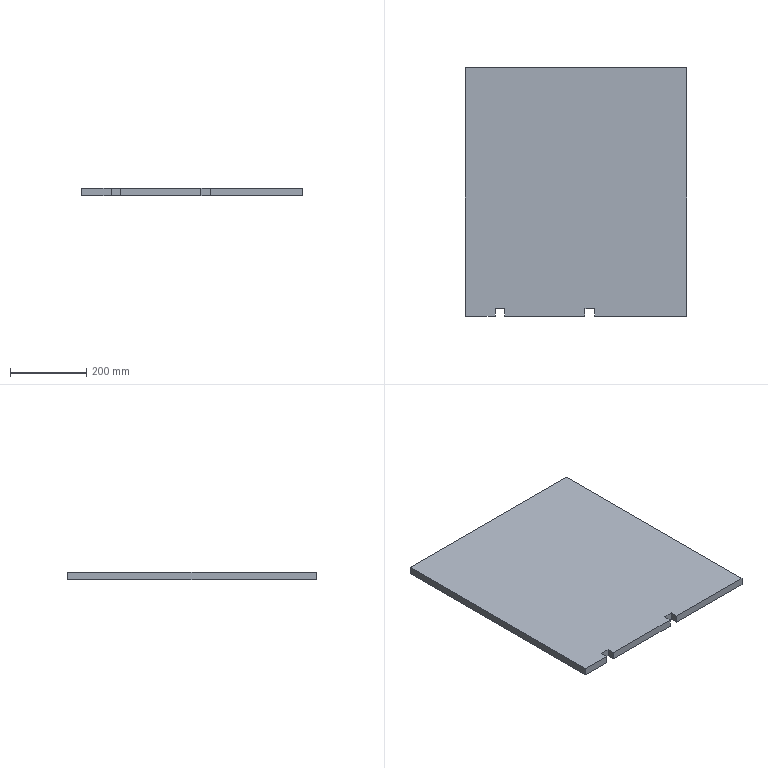Component | SolidWorks | ElectromagneticBeamBasePlate2-1 | 1 solid | 14 faces | box 579 x 650 x 20 mm | volume 7507000 mm3 | plane 14 | material Plain Carbon Steel
STEP:
#1=COLOUR_RGB('',0.7922,0.8196,0.9333);
#2=FILL_AREA_STYLE_COLOUR('',#1);
#3=FILL_AREA_STYLE('',(#2));
#4=SURFACE_STYLE_FILL_AREA(#3);
#5=SURFACE_SIDE_STYLE('',(#4));
#6=SURFACE_STYLE_USAGE(.BOTH.,#5);
#7=PRESENTATION_STYLE_ASSIGNMENT((#6));
#8=CARTESIAN_POINT('',(-258.877,140.226,239.923));
#9=VERTEX_POINT('',#8);
#10=CARTESIAN_POINT('',(-258.877,114.635,239.923));
#11=VERTEX_POINT('',#10);
#12=CARTESIAN_POINT('',(-258.877,140.226,239.923));
#13=DIRECTION('',(0.,-1.,-0.));
#14=VECTOR('',#13,39.37);
#15=LINE('',#12,#14);
#16=EDGE_CURVE('',#9,#11,#15,.T.);
#17=ORIENTED_EDGE('',*,*,#16,.F.);
#18=CARTESIAN_POINT('',(-258.877,140.226,239.136));
#19=VERTEX_POINT('',#18);
#20=CARTESIAN_POINT('',(-258.877,140.226,239.136));
#21=DIRECTION('',(0.,-0.,1.));
#22=VECTOR('',#21,39.37);
#23=LINE('',#20,#22);
#24=EDGE_CURVE('',#19,#9,#23,.T.);
#25=ORIENTED_EDGE('',*,*,#24,.F.);
#26=CARTESIAN_POINT('',(-258.877,114.635,239.136));
#27=VERTEX_POINT('',#26);
#28=CARTESIAN_POINT('',(-258.877,140.226,239.136));
#29=DIRECTION('',(0.,-1.,-0.));
#30=VECTOR('',#29,39.37);
#31=LINE('',#28,#30);
#32=EDGE_CURVE('',#19,#27,#31,.T.);
#33=ORIENTED_EDGE('',*,*,#32,.T.);
#34=CARTESIAN_POINT('',(-258.877,114.635,239.136));
#35=DIRECTION('',(0.,-0.,1.));
#36=VECTOR('',#35,39.37);
#37=LINE('',#34,#36);
#38=EDGE_CURVE('',#27,#11,#37,.T.);
#39=ORIENTED_EDGE('',*,*,#38,.T.);
#40=EDGE_LOOP('',(#17,#25,#33,#39));
#41=FACE_OUTER_BOUND('',#40,.T.);
#42=CARTESIAN_POINT('',(-258.877,140.226,239.136));
#43=DIRECTION('',(-1.,-0.,-0.));
#44=DIRECTION('',(0.,-1.,-0.));
#45=AXIS2_PLACEMENT_3D('',#42,#43,#44);
#46=PLANE('',#45);
#47=ADVANCED_FACE('',(#41),#46,.T.);
#48=CARTESIAN_POINT('',(-236.081,140.226,239.923));
#49=VERTEX_POINT('',#48);
#50=CARTESIAN_POINT('',(-258.877,140.226,239.923));
#51=DIRECTION('',(-1.,0.,0.));
#52=VECTOR('',#51,39.37);
#53=LINE('',#50,#52);
#54=EDGE_CURVE('',#49,#9,#53,.T.);
#55=ORIENTED_EDGE('',*,*,#54,.F.);
#56=CARTESIAN_POINT('',(-236.081,140.226,239.136));
#57=VERTEX_POINT('',#56);
#58=CARTESIAN_POINT('',(-236.081,140.226,239.136));
#59=DIRECTION('',(0.,-0.,1.));
#60=VECTOR('',#59,39.37);
#61=LINE('',#58,#60);
#62=EDGE_CURVE('',#57,#49,#61,.T.);
#63=ORIENTED_EDGE('',*,*,#62,.F.);
#64=CARTESIAN_POINT('',(-258.877,140.226,239.136));
#65=DIRECTION('',(-1.,0.,0.));
#66=VECTOR('',#65,39.37);
#67=LINE('',#64,#66);
#68=EDGE_CURVE('',#57,#19,#67,.T.);
#69=ORIENTED_EDGE('',*,*,#68,.T.);
#70=ORIENTED_EDGE('',*,*,#24,.T.);
#71=EDGE_LOOP('',(#55,#63,#69,#70));
#72=FACE_OUTER_BOUND('',#71,.T.);
#73=CARTESIAN_POINT('',(-258.877,140.226,239.136));
#74=DIRECTION('',(0.,1.,0.));
#75=DIRECTION('',(-1.,0.,0.));
#76=AXIS2_PLACEMENT_3D('',#73,#74,#75);
#77=PLANE('',#76);
#78=ADVANCED_FACE('',(#72),#77,.T.);
#79=CARTESIAN_POINT('',(-236.081,114.635,239.923));
#80=VERTEX_POINT('',#79);
#81=CARTESIAN_POINT('',(-236.081,140.226,239.923));
#82=DIRECTION('',(-0.,1.,0.));
#83=VECTOR('',#82,39.37);
#84=LINE('',#81,#83);
#85=EDGE_CURVE('',#80,#49,#84,.T.);
#86=ORIENTED_EDGE('',*,*,#85,.F.);
#87=CARTESIAN_POINT('',(-236.081,114.635,239.136));
#88=VERTEX_POINT('',#87);
#89=CARTESIAN_POINT('',(-236.081,114.635,239.136));
#90=DIRECTION('',(0.,-0.,1.));
#91=VECTOR('',#90,39.37);
#92=LINE('',#89,#91);
#93=EDGE_CURVE('',#88,#80,#92,.T.);
#94=ORIENTED_EDGE('',*,*,#93,.F.);
#95=CARTESIAN_POINT('',(-236.081,140.226,239.136));
#96=DIRECTION('',(-0.,1.,0.));
#97=VECTOR('',#96,39.37);
#98=LINE('',#95,#97);
#99=EDGE_CURVE('',#88,#57,#98,.T.);
#100=ORIENTED_EDGE('',*,*,#99,.T.);
#101=ORIENTED_EDGE('',*,*,#62,.T.);
#102=EDGE_LOOP('',(#86,#94,#100,#101));
#103=FACE_OUTER_BOUND('',#102,.T.);
#104=CARTESIAN_POINT('',(-236.081,140.226,239.136));
#105=DIRECTION('',(1.,0.,0.));
#106=DIRECTION('',(-0.,1.,0.));
#107=AXIS2_PLACEMENT_3D('',#104,#105,#106);
#108=PLANE('',#107);
#109=ADVANCED_FACE('',(#103),#108,.T.);
#110=CARTESIAN_POINT('',(-245.569,114.635,239.923));
#111=VERTEX_POINT('',#110);
#112=CARTESIAN_POINT('',(-245.569,114.635,239.923));
#113=DIRECTION('',(1.,0.,0.));
#114=VECTOR('',#113,39.37);
#115=LINE('',#112,#114);
#116=EDGE_CURVE('',#111,#80,#115,.T.);
#117=ORIENTED_EDGE('',*,*,#116,.F.);
#118=CARTESIAN_POINT('',(-245.569,114.635,239.136));
#119=VERTEX_POINT('',#118);
#120=CARTESIAN_POINT('',(-245.569,114.635,239.136));
#121=DIRECTION('',(0.,-0.,1.));
#122=VECTOR('',#121,39.37);
#123=LINE('',#120,#122);
#124=EDGE_CURVE('',#119,#111,#123,.T.);
#125=ORIENTED_EDGE('',*,*,#124,.F.);
#126=CARTESIAN_POINT('',(-245.569,114.635,239.136));
#127=DIRECTION('',(1.,0.,0.));
#128=VECTOR('',#127,39.37);
#129=LINE('',#126,#128);
#130=EDGE_CURVE('',#119,#88,#129,.T.);
#131=ORIENTED_EDGE('',*,*,#130,.T.);
#132=ORIENTED_EDGE('',*,*,#93,.T.);
#133=EDGE_LOOP('',(#117,#125,#131,#132));
#134=FACE_OUTER_BOUND('',#133,.T.);
#135=CARTESIAN_POINT('',(-245.569,114.635,239.136));
#136=DIRECTION('',(0.,-1.,-0.));
#137=DIRECTION('',(1.,0.,0.));
#138=AXIS2_PLACEMENT_3D('',#135,#136,#137);
#139=PLANE('',#138);
#140=ADVANCED_FACE('',(#134),#139,.T.);
#141=CARTESIAN_POINT('',(-245.569,115.423,239.923));
#142=VERTEX_POINT('',#141);
#143=CARTESIAN_POINT('',(-245.569,115.423,239.923));
#144=DIRECTION('',(0.,-1.,-0.));
#145=VECTOR('',#144,39.37);
#146=LINE('',#143,#145);
#147=EDGE_CURVE('',#142,#111,#146,.T.);
#148=ORIENTED_EDGE('',*,*,#147,.F.);
#149=CARTESIAN_POINT('',(-245.569,115.423,239.136));
#150=VERTEX_POINT('',#149);
#151=CARTESIAN_POINT('',(-245.569,115.423,239.136));
#152=DIRECTION('',(0.,-0.,1.));
#153=VECTOR('',#152,39.37);
#154=LINE('',#151,#153);
#155=EDGE_CURVE('',#150,#142,#154,.T.);
#156=ORIENTED_EDGE('',*,*,#155,.F.);
#157=CARTESIAN_POINT('',(-245.569,115.423,239.136));
#158=DIRECTION('',(0.,-1.,-0.));
#159=VECTOR('',#158,39.37);
#160=LINE('',#157,#159);
#161=EDGE_CURVE('',#150,#119,#160,.T.);
#162=ORIENTED_EDGE('',*,*,#161,.T.);
#163=ORIENTED_EDGE('',*,*,#124,.T.);
#164=EDGE_LOOP('',(#148,#156,#162,#163));
#165=FACE_OUTER_BOUND('',#164,.T.);
#166=CARTESIAN_POINT('',(-245.569,115.423,239.136));
#167=DIRECTION('',(-1.,0.,0.));
#168=DIRECTION('',(0.,-1.,-0.));
#169=AXIS2_PLACEMENT_3D('',#166,#167,#168);
#170=PLANE('',#169);
#171=ADVANCED_FACE('',(#165),#170,.T.);
#172=CARTESIAN_POINT('',(-246.554,115.423,239.923));
#173=VERTEX_POINT('',#172);
#174=CARTESIAN_POINT('',(-246.554,115.423,239.923));
#175=DIRECTION('',(1.,0.,0.));
#176=VECTOR('',#175,39.37);
#177=LINE('',#174,#176);
#178=EDGE_CURVE('',#173,#142,#177,.T.);
#179=ORIENTED_EDGE('',*,*,#178,.F.);
#180=CARTESIAN_POINT('',(-246.554,115.423,239.136));
#181=VERTEX_POINT('',#180);
#182=CARTESIAN_POINT('',(-246.554,115.423,239.136));
#183=DIRECTION('',(0.,-0.,1.));
#184=VECTOR('',#183,39.37);
#185=LINE('',#182,#184);
#186=EDGE_CURVE('',#181,#173,#185,.T.);
#187=ORIENTED_EDGE('',*,*,#186,.F.);
#188=CARTESIAN_POINT('',(-246.554,115.423,239.136));
#189=DIRECTION('',(1.,0.,0.));
#190=VECTOR('',#189,39.37);
#191=LINE('',#188,#190);
#192=EDGE_CURVE('',#181,#150,#191,.T.);
#193=ORIENTED_EDGE('',*,*,#192,.T.);
#194=ORIENTED_EDGE('',*,*,#155,.T.);
#195=EDGE_LOOP('',(#179,#187,#193,#194));
#196=FACE_OUTER_BOUND('',#195,.T.);
#197=CARTESIAN_POINT('',(-246.554,115.423,239.136));
#198=DIRECTION('',(0.,-1.,-0.));
#199=DIRECTION('',(1.,0.,0.));
#200=AXIS2_PLACEMENT_3D('',#197,#198,#199);
#201=PLANE('',#200);
#202=ADVANCED_FACE('',(#196),#201,.T.);
#203=CARTESIAN_POINT('',(-246.554,114.635,239.923));
#204=VERTEX_POINT('',#203);
#205=CARTESIAN_POINT('',(-246.554,114.635,239.923));
#206=DIRECTION('',(0.,1.,0.));
#207=VECTOR('',#206,39.37);
#208=LINE('',#205,#207);
#209=EDGE_CURVE('',#204,#173,#208,.T.);
#210=ORIENTED_EDGE('',*,*,#209,.F.);
#211=CARTESIAN_POINT('',(-246.554,114.635,239.136));
#212=VERTEX_POINT('',#211);
#213=CARTESIAN_POINT('',(-246.554,114.635,239.136));
#214=DIRECTION('',(0.,-0.,1.));
#215=VECTOR('',#214,39.37);
#216=LINE('',#213,#215);
#217=EDGE_CURVE('',#212,#204,#216,.T.);
#218=ORIENTED_EDGE('',*,*,#217,.F.);
#219=CARTESIAN_POINT('',(-246.554,114.635,239.136));
#220=DIRECTION('',(0.,1.,0.));
#221=VECTOR('',#220,39.37);
#222=LINE('',#219,#221);
#223=EDGE_CURVE('',#212,#181,#222,.T.);
#224=ORIENTED_EDGE('',*,*,#223,.T.);
#225=ORIENTED_EDGE('',*,*,#186,.T.);
#226=EDGE_LOOP('',(#210,#218,#224,#225));
#227=FACE_OUTER_BOUND('',#226,.T.);
#228=CARTESIAN_POINT('',(-246.554,114.635,239.136));
#229=DIRECTION('',(1.,0.,0.));
#230=DIRECTION('',(0.,1.,0.));
#231=AXIS2_PLACEMENT_3D('',#228,#229,#230);
#232=PLANE('',#231);
#233=ADVANCED_FACE('',(#227),#232,.T.);
#234=CARTESIAN_POINT('',(-254.821,114.635,239.923));
#235=VERTEX_POINT('',#234);
#236=CARTESIAN_POINT('',(-254.821,114.635,239.923));
#237=DIRECTION('',(1.,0.,0.));
#238=VECTOR('',#237,39.37);
#239=LINE('',#236,#238);
#240=EDGE_CURVE('',#235,#204,#239,.T.);
#241=ORIENTED_EDGE('',*,*,#240,.F.);
#242=CARTESIAN_POINT('',(-254.821,114.635,239.136));
#243=VERTEX_POINT('',#242);
#244=CARTESIAN_POINT('',(-254.821,114.635,239.136));
#245=DIRECTION('',(0.,-0.,1.));
#246=VECTOR('',#245,39.37);
#247=LINE('',#244,#246);
#248=EDGE_CURVE('',#243,#235,#247,.T.);
#249=ORIENTED_EDGE('',*,*,#248,.F.);
#250=CARTESIAN_POINT('',(-254.821,114.635,239.136));
#251=DIRECTION('',(1.,0.,0.));
#252=VECTOR('',#251,39.37);
#253=LINE('',#250,#252);
#254=EDGE_CURVE('',#243,#212,#253,.T.);
#255=ORIENTED_EDGE('',*,*,#254,.T.);
#256=ORIENTED_EDGE('',*,*,#217,.T.);
#257=EDGE_LOOP('',(#241,#249,#255,#256));
#258=FACE_OUTER_BOUND('',#257,.T.);
#259=CARTESIAN_POINT('',(-254.821,114.635,239.136));
#260=DIRECTION('',(0.,-1.,-0.));
#261=DIRECTION('',(1.,0.,0.));
#262=AXIS2_PLACEMENT_3D('',#259,#260,#261);
#263=PLANE('',#262);
#264=ADVANCED_FACE('',(#258),#263,.T.);
#265=CARTESIAN_POINT('',(-254.821,115.423,239.923));
#266=VERTEX_POINT('',#265);
#267=CARTESIAN_POINT('',(-254.821,115.423,239.923));
#268=DIRECTION('',(0.,-1.,-0.));
#269=VECTOR('',#268,39.37);
#270=LINE('',#267,#269);
#271=EDGE_CURVE('',#266,#235,#270,.T.);
#272=ORIENTED_EDGE('',*,*,#271,.F.);
#273=CARTESIAN_POINT('',(-254.821,115.423,239.136));
#274=VERTEX_POINT('',#273);
#275=CARTESIAN_POINT('',(-254.821,115.423,239.136));
#276=DIRECTION('',(0.,-0.,1.));
#277=VECTOR('',#276,39.37);
#278=LINE('',#275,#277);
#279=EDGE_CURVE('',#274,#266,#278,.T.);
#280=ORIENTED_EDGE('',*,*,#279,.F.);
#281=CARTESIAN_POINT('',(-254.821,115.423,239.136));
#282=DIRECTION('',(0.,-1.,-0.));
#283=VECTOR('',#282,39.37);
#284=LINE('',#281,#283);
#285=EDGE_CURVE('',#274,#243,#284,.T.);
#286=ORIENTED_EDGE('',*,*,#285,.T.);
#287=ORIENTED_EDGE('',*,*,#248,.T.);
#288=EDGE_LOOP('',(#272,#280,#286,#287));
#289=FACE_OUTER_BOUND('',#288,.T.);
#290=CARTESIAN_POINT('',(-254.821,115.423,239.136));
#291=DIRECTION('',(-1.,0.,0.));
#292=DIRECTION('',(0.,-1.,-0.));
#293=AXIS2_PLACEMENT_3D('',#290,#291,#292);
#294=PLANE('',#293);
#295=ADVANCED_FACE('',(#289),#294,.T.);
#296=CARTESIAN_POINT('',(-255.806,115.423,239.923));
#297=VERTEX_POINT('',#296);
#298=CARTESIAN_POINT('',(-255.806,115.423,239.923));
#299=DIRECTION('',(1.,0.,0.));
#300=VECTOR('',#299,39.37);
#301=LINE('',#298,#300);
#302=EDGE_CURVE('',#297,#266,#301,.T.);
#303=ORIENTED_EDGE('',*,*,#302,.F.);
#304=CARTESIAN_POINT('',(-255.806,115.423,239.136));
#305=VERTEX_POINT('',#304);
#306=CARTESIAN_POINT('',(-255.806,115.423,239.136));
#307=DIRECTION('',(0.,-0.,1.));
#308=VECTOR('',#307,39.37);
#309=LINE('',#306,#308);
#310=EDGE_CURVE('',#305,#297,#309,.T.);
#311=ORIENTED_EDGE('',*,*,#310,.F.);
#312=CARTESIAN_POINT('',(-255.806,115.423,239.136));
#313=DIRECTION('',(1.,0.,0.));
#314=VECTOR('',#313,39.37);
#315=LINE('',#312,#314);
#316=EDGE_CURVE('',#305,#274,#315,.T.);
#317=ORIENTED_EDGE('',*,*,#316,.T.);
#318=ORIENTED_EDGE('',*,*,#279,.T.);
#319=EDGE_LOOP('',(#303,#311,#317,#318));
#320=FACE_OUTER_BOUND('',#319,.T.);
#321=CARTESIAN_POINT('',(-255.806,115.423,239.136));
#322=DIRECTION('',(0.,-1.,-0.));
#323=DIRECTION('',(1.,0.,0.));
#324=AXIS2_PLACEMENT_3D('',#321,#322,#323);
#325=PLANE('',#324);
#326=ADVANCED_FACE('',(#320),#325,.T.);
#327=CARTESIAN_POINT('',(-255.806,114.635,239.923));
#328=VERTEX_POINT('',#327);
#329=CARTESIAN_POINT('',(-255.806,114.635,239.923));
#330=DIRECTION('',(0.,1.,0.));
#331=VECTOR('',#330,39.37);
#332=LINE('',#329,#331);
#333=EDGE_CURVE('',#328,#297,#332,.T.);
#334=ORIENTED_EDGE('',*,*,#333,.F.);
#335=CARTESIAN_POINT('',(-255.806,114.635,239.136));
#336=VERTEX_POINT('',#335);
#337=CARTESIAN_POINT('',(-255.806,114.635,239.136));
#338=DIRECTION('',(0.,-0.,1.));
#339=VECTOR('',#338,39.37);
#340=LINE('',#337,#339);
#341=EDGE_CURVE('',#336,#328,#340,.T.);
#342=ORIENTED_EDGE('',*,*,#341,.F.);
#343=CARTESIAN_POINT('',(-255.806,114.635,239.136));
#344=DIRECTION('',(0.,1.,0.));
#345=VECTOR('',#344,39.37);
#346=LINE('',#343,#345);
#347=EDGE_CURVE('',#336,#305,#346,.T.);
#348=ORIENTED_EDGE('',*,*,#347,.T.);
#349=ORIENTED_EDGE('',*,*,#310,.T.);
#350=EDGE_LOOP('',(#334,#342,#348,#349));
#351=FACE_OUTER_BOUND('',#350,.T.);
#352=CARTESIAN_POINT('',(-255.806,114.635,239.136));
#353=DIRECTION('',(1.,0.,0.));
#354=DIRECTION('',(0.,1.,0.));
#355=AXIS2_PLACEMENT_3D('',#352,#353,#354);
#356=PLANE('',#355);
#357=ADVANCED_FACE('',(#351),#356,.T.);
#358=CARTESIAN_POINT('',(-258.877,114.635,239.923));
#359=DIRECTION('',(1.,0.,0.));
#360=VECTOR('',#359,39.37);
#361=LINE('',#358,#360);
#362=EDGE_CURVE('',#11,#328,#361,.T.);
#363=ORIENTED_EDGE('',*,*,#362,.F.);
#364=ORIENTED_EDGE('',*,*,#38,.F.);
#365=CARTESIAN_POINT('',(-258.877,114.635,239.136));
#366=DIRECTION('',(1.,0.,0.));
#367=VECTOR('',#366,39.37);
#368=LINE('',#365,#367);
#369=EDGE_CURVE('',#27,#336,#368,.T.);
#370=ORIENTED_EDGE('',*,*,#369,.T.);
#371=ORIENTED_EDGE('',*,*,#341,.T.);
#372=EDGE_LOOP('',(#363,#364,#370,#371));
#373=FACE_OUTER_BOUND('',#372,.T.);
#374=CARTESIAN_POINT('',(-258.877,114.635,239.136));
#375=DIRECTION('',(0.,-1.,-0.));
#376=DIRECTION('',(1.,0.,0.));
#377=AXIS2_PLACEMENT_3D('',#374,#375,#376);
#378=PLANE('',#377);
#379=ADVANCED_FACE('',(#373),#378,.T.);
#380=ORIENTED_EDGE('',*,*,#32,.F.);
#381=ORIENTED_EDGE('',*,*,#68,.F.);
#382=ORIENTED_EDGE('',*,*,#99,.F.);
#383=ORIENTED_EDGE('',*,*,#130,.F.);
#384=ORIENTED_EDGE('',*,*,#161,.F.);
#385=ORIENTED_EDGE('',*,*,#192,.F.);
#386=ORIENTED_EDGE('',*,*,#223,.F.);
#387=ORIENTED_EDGE('',*,*,#254,.F.);
#388=ORIENTED_EDGE('',*,*,#285,.F.);
#389=ORIENTED_EDGE('',*,*,#316,.F.);
#390=ORIENTED_EDGE('',*,*,#347,.F.);
#391=ORIENTED_EDGE('',*,*,#369,.F.);
#392=EDGE_LOOP('',(#380,#381,#382,#383,#384,#385,#386,#387,#388,#389,#390,#391));
#393=FACE_OUTER_BOUND('',#392,.T.);
#394=CARTESIAN_POINT('',(-258.877,140.226,239.136));
#395=DIRECTION('',(0.,-0.,1.));
#396=DIRECTION('',(0.,-1.,-0.));
#397=AXIS2_PLACEMENT_3D('',#394,#395,#396);
#398=PLANE('',#397);
#399=ADVANCED_FACE('',(#393),#398,.F.);
#400=ORIENTED_EDGE('',*,*,#16,.T.);
#401=ORIENTED_EDGE('',*,*,#362,.T.);
#402=ORIENTED_EDGE('',*,*,#333,.T.);
#403=ORIENTED_EDGE('',*,*,#302,.T.);
#404=ORIENTED_EDGE('',*,*,#271,.T.);
#405=ORIENTED_EDGE('',*,*,#240,.T.);
#406=ORIENTED_EDGE('',*,*,#209,.T.);
#407=ORIENTED_EDGE('',*,*,#178,.T.);
#408=ORIENTED_EDGE('',*,*,#147,.T.);
#409=ORIENTED_EDGE('',*,*,#116,.T.);
#410=ORIENTED_EDGE('',*,*,#85,.T.);
#411=ORIENTED_EDGE('',*,*,#54,.T.);
#412=EDGE_LOOP('',(#400,#401,#402,#403,#404,#405,#406,#407,#408,#409,#410,#411));
#413=FACE_OUTER_BOUND('',#412,.T.);
#414=CARTESIAN_POINT('',(-258.877,140.226,239.923));
#415=DIRECTION('',(0.,-0.,1.));
#416=DIRECTION('',(0.,-1.,-0.));
#417=AXIS2_PLACEMENT_3D('',#414,#415,#416);
#418=PLANE('',#417);
#419=ADVANCED_FACE('',(#413),#418,.T.);
#420=CLOSED_SHELL('',(#47,#78,#109,#140,#171,#202,#233,#264,#295,#326,#357,#379,#399,#419));
#421=MANIFOLD_SOLID_BREP('',#420);
#422=STYLED_ITEM('',(#7),#421);
#423=(LENGTH_UNIT()NAMED_UNIT(*)SI_UNIT($,.METRE.));
#424=LENGTH_MEASURE_WITH_UNIT(LENGTH_MEASURE(0.0254),#423);
#425=DIMENSIONAL_EXPONENTS(1.,0.,0.,0.,0.,0.,0.);
#426=(CONVERSION_BASED_UNIT('',#424)LENGTH_UNIT()NAMED_UNIT(#425));
#427=UNCERTAINTY_MEASURE_WITH_UNIT(LENGTH_MEASURE(0.00001),#426,'','');
#428=(NAMED_UNIT(*)PLANE_ANGLE_UNIT()SI_UNIT($,.RADIAN.));
#429=(NAMED_UNIT(*)SI_UNIT($,.STERADIAN.)SOLID_ANGLE_UNIT());
#430=(GEOMETRIC_REPRESENTATION_CONTEXT(3)GLOBAL_UNCERTAINTY_ASSIGNED_CONTEXT((#427))GLOBAL_UNIT_ASSIGNED_CONTEXT((#426,#428,#429))REPRESENTATION_CONTEXT('',''));
#431=MECHANICAL_DESIGN_GEOMETRIC_PRESENTATION_REPRESENTATION('',(#422),#430);
#432=PRESENTATION_LAYER_ASSIGNMENT('','',(#422));
#433=CARTESIAN_POINT('',(0.,0.,0.));
#434=DIRECTION('',(0.,0.,1.));
#435=DIRECTION('',(1.,0.,0.));
#436=AXIS2_PLACEMENT_3D('',#433,#434,#435);
#437=(LENGTH_UNIT()NAMED_UNIT(*)SI_UNIT($,.METRE.));
#438=LENGTH_MEASURE_WITH_UNIT(LENGTH_MEASURE(0.0254),#437);
#439=DIMENSIONAL_EXPONENTS(1.,0.,0.,0.,0.,0.,0.);
#440=(CONVERSION_BASED_UNIT('',#438)LENGTH_UNIT()NAMED_UNIT(#439));
#441=UNCERTAINTY_MEASURE_WITH_UNIT(LENGTH_MEASURE(0.00001),#440,'','');
#442=(NAMED_UNIT(*)PLANE_ANGLE_UNIT()SI_UNIT($,.RADIAN.));
#443=(NAMED_UNIT(*)SI_UNIT($,.STERADIAN.)SOLID_ANGLE_UNIT());
#444=(GEOMETRIC_REPRESENTATION_CONTEXT(3)GLOBAL_UNCERTAINTY_ASSIGNED_CONTEXT((#441))GLOBAL_UNIT_ASSIGNED_CONTEXT((#440,#442,#443))REPRESENTATION_CONTEXT('',''));
#445=ADVANCED_BREP_SHAPE_REPRESENTATION('',(#421,#436),#444);